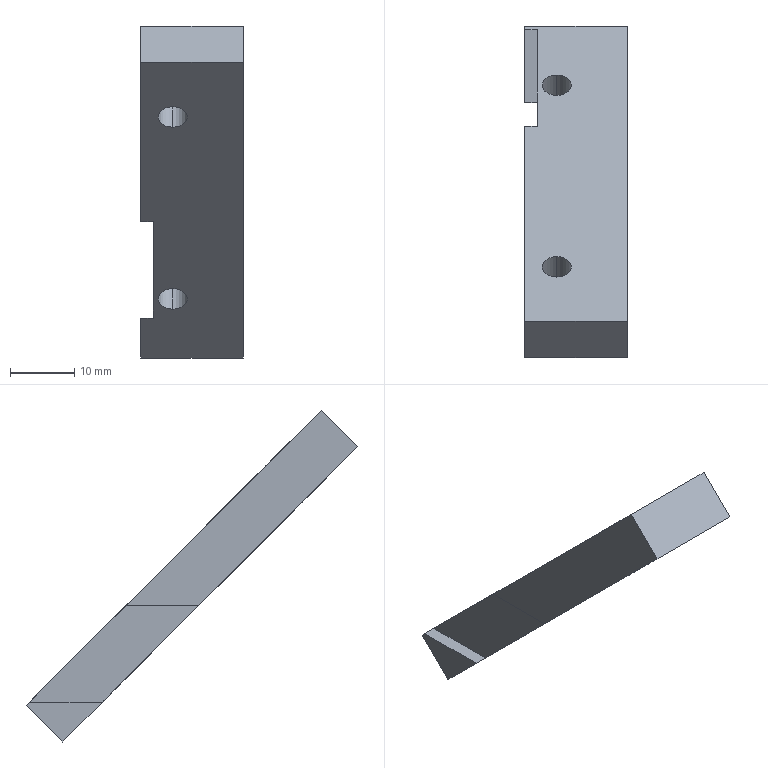Component | SolidWorks | ZL-10-04LeftCoverPlate-1 | 1 solid | 14 faces | box 16 x 51.62 x 51.62 mm | volume 7726 mm3 | plane 10 | cylinder 4 | commonest cylinder face diameters 4.5 x4
build123d program:
from build123d import *

# Parameters (mm, degrees)
SKETCH1_W          = 16
SKETCH1_H          = 65
EXTRUDE1_DEPTH     = 4
SKETCH2_R          = 2.25
CUT_EXTRUDE1_DEPTH = 66.977
CUT_EXTRUDE2_DEPTH = 2


with BuildPart() as part:
    # Sketch1 → Extrude1 (new, symmetric)
    with BuildSketch(Plane(origin=(0, 0, 0), x_dir=(1, 0, 0), z_dir=(0, 1, 0))):
        with Locations((0, 32.5)):
            Rectangle(SKETCH1_W, SKETCH1_H)
    extrude(amount=EXTRUDE1_DEPTH, both=True)

    # Sketch2 → Cut-Extrude1 (cut, through all)
    with BuildSketch(Plane(origin=(0, 4, 0), x_dir=(1, 0, 0), z_dir=(0, 1, 0))):
        with Locations(Location((-3, 12, 0), (0, 0, 270))):
            Circle(SKETCH2_R)
        with Locations(Location((-3, 52, 0), (0, 0, 270))):
            Circle(SKETCH2_R)
    extrude(amount=-CUT_EXTRUDE1_DEPTH, mode=Mode.SUBTRACT)

    # Sketch3 → Cut-Extrude2 (cut)
    with BuildSketch(Plane.ZY.offset(8)):
        Polygon((-43, 4), (-35, -4), (-56.213, -4), (-64.213, 4), align=None)
    extrude(amount=-CUT_EXTRUDE2_DEPTH, mode=Mode.SUBTRACT)


solid = part.part

# Placed as in the assembly
solid = solid.moved(Location((30.823, 52.714, 18.077), (45, 0, 0)))